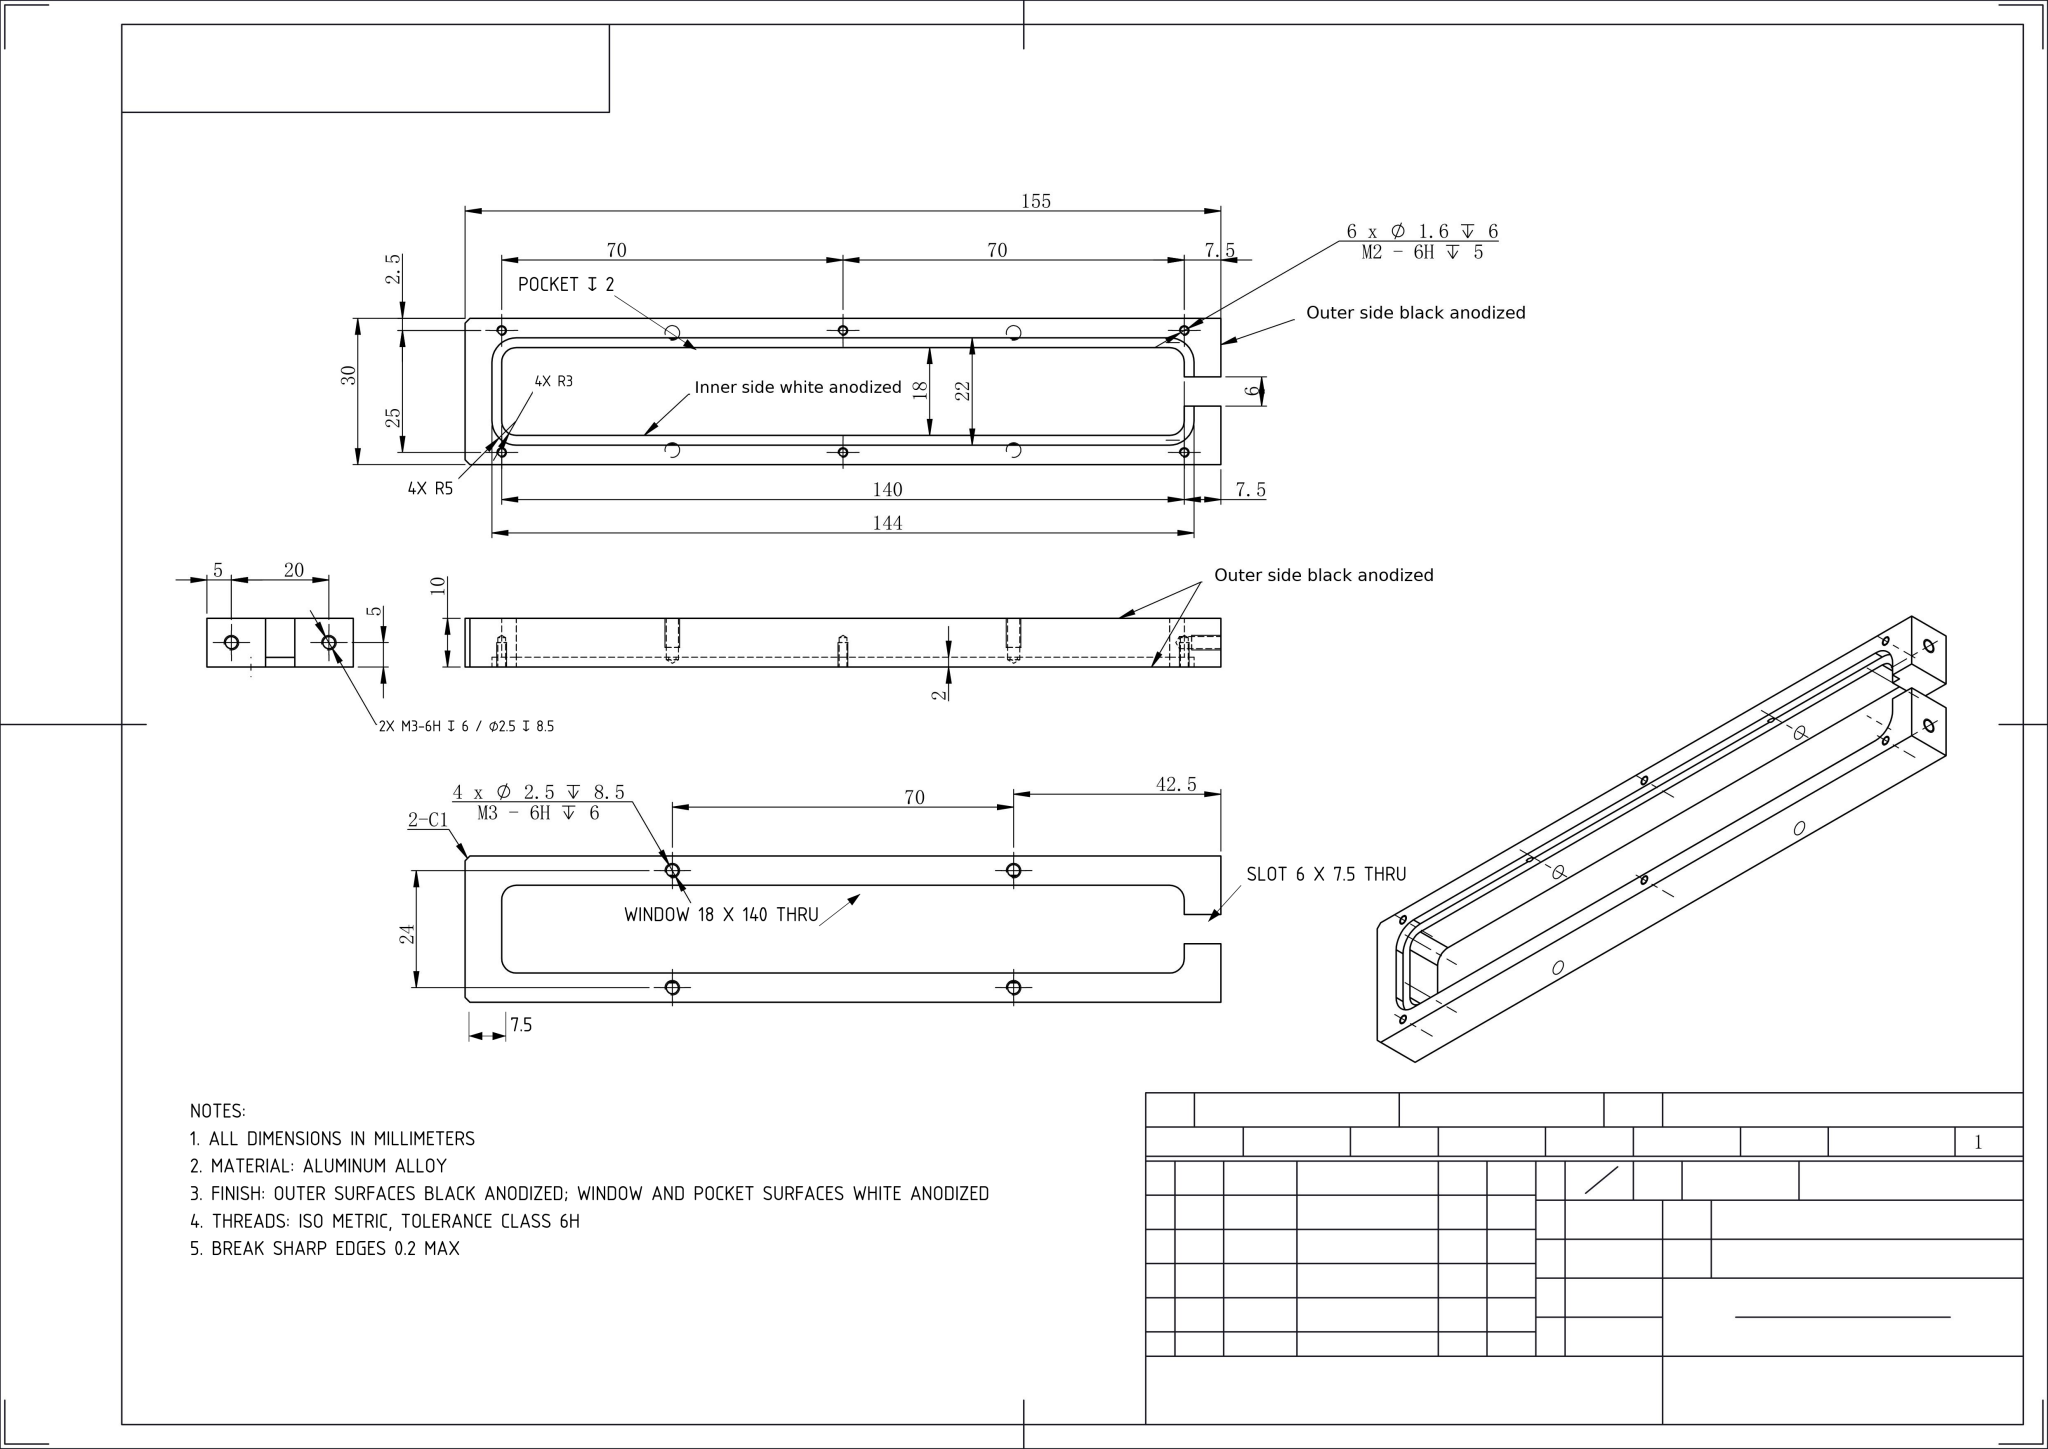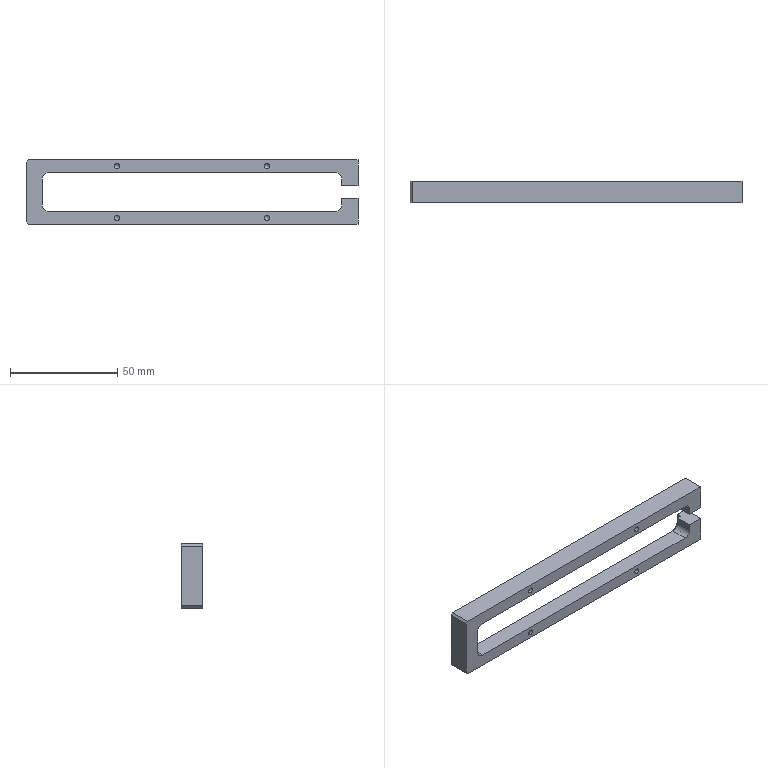Part | NX | mm | Rectangular U-Channel Frame Panel 155mm | 1 solid | 78 faces | box 155 x 10 x 30 mm | volume 19341 mm3 | cylinder 32 | cone 24 | plane 22 | commonest cylinder face diameters 2.5 x12 1.6 x12 10 x4 6 x4